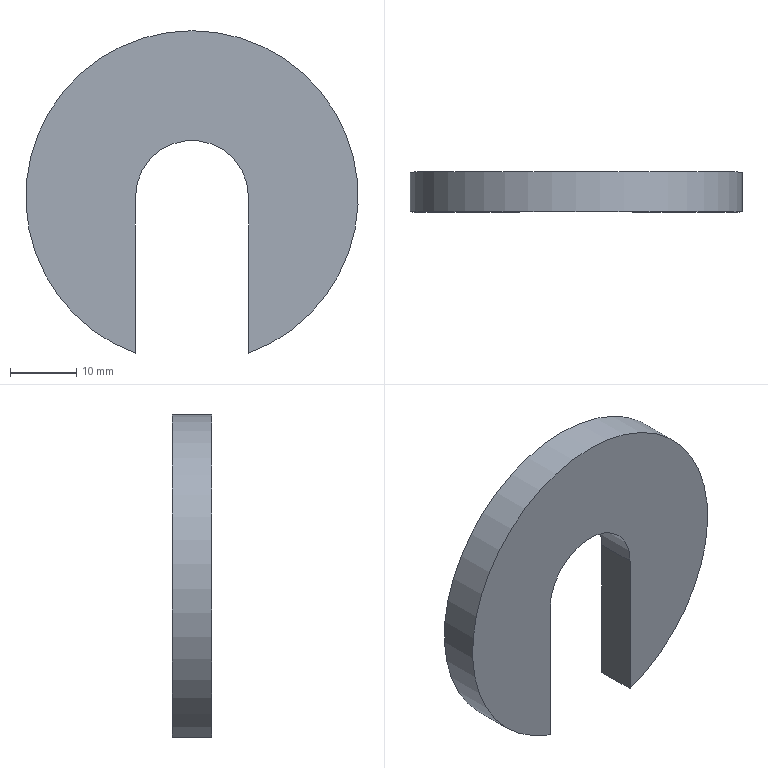Component | NX | C_WASHER | 1 solid | 6 faces | box 50 x 6 x 48.51 mm | volume 8600 mm3 | plane 4 | cylinder 2 | commonest cylinder face diameters 17 x1 50 x1
STEP:
#1=CARTESIAN_POINT('',(0.,0.,0.));
#2=DIRECTION('',(0.,0.,1.));
#3=DIRECTION('',(1.,0.,0.));
#4=AXIS2_PLACEMENT_3D('',#1,#2,#3);
#5=CARTESIAN_POINT('',(-8.5,-38.,42.489));
#6=VERTEX_POINT('',#5);
#7=CARTESIAN_POINT('',(-8.5,-38.,66.));
#8=VERTEX_POINT('',#7);
#9=CARTESIAN_POINT('',(-8.5,-38.,42.489));
#10=DIRECTION('',(-0.,0.,1.));
#11=VECTOR('',#10,1.);
#12=LINE('',#9,#11);
#13=CARTESIAN_POINT('',(-8.5,-44.,42.489));
#14=DIRECTION('',(-1.,0.,-0.));
#15=DIRECTION('',(0.,0.,-1.));
#16=AXIS2_PLACEMENT_3D('',#13,#14,#15);
#17=PLANE('',#16);
#18=CARTESIAN_POINT('',(0.,-6.));
#19=DIRECTION('',(-1.,0.));
#20=VECTOR('',#19,1.);
#21=LINE('',#18,#20);
#22=(GEOMETRIC_REPRESENTATION_CONTEXT(2)PARAMETRIC_REPRESENTATION_CONTEXT()REPRESENTATION_CONTEXT('',''));
#23=DEFINITIONAL_REPRESENTATION('',(#21),#22);
#24=PCURVE('',#17,#23);
#25=CARTESIAN_POINT('',(0.,-38.,66.));
#26=DIRECTION('',(0.,1.,0.));
#27=DIRECTION('',(0.,0.,1.));
#28=AXIS2_PLACEMENT_3D('',#25,#26,#27);
#29=PLANE('',#28);
#30=CARTESIAN_POINT('',(-23.511,-8.5));
#31=DIRECTION('',(1.,-0.));
#32=VECTOR('',#31,1.);
#33=LINE('',#30,#32);
#34=(GEOMETRIC_REPRESENTATION_CONTEXT(2)PARAMETRIC_REPRESENTATION_CONTEXT()REPRESENTATION_CONTEXT('',''));
#35=DEFINITIONAL_REPRESENTATION('',(#33),#34);
#36=PCURVE('',#29,#35);
#37=SURFACE_CURVE('',#12,(#24,#36),.PCURVE_S1.);
#38=EDGE_CURVE('',#6,#8,#37,.T.);
#39=ORIENTED_EDGE('',*,*,#38,.T.);
#40=CARTESIAN_POINT('',(-8.5,-44.,66.));
#41=VERTEX_POINT('',#40);
#42=CARTESIAN_POINT('',(-8.5,-44.,66.));
#43=DIRECTION('',(0.,1.,0.));
#44=VECTOR('',#43,1.);
#45=LINE('',#42,#44);
#46=CARTESIAN_POINT('',(-23.511,0.));
#47=DIRECTION('',(0.,-1.));
#48=VECTOR('',#47,1.);
#49=LINE('',#46,#48);
#50=(GEOMETRIC_REPRESENTATION_CONTEXT(2)PARAMETRIC_REPRESENTATION_CONTEXT()REPRESENTATION_CONTEXT('',''));
#51=DEFINITIONAL_REPRESENTATION('',(#49),#50);
#52=PCURVE('',#17,#51);
#53=CARTESIAN_POINT('',(0.,-44.,66.));
#54=DIRECTION('',(0.,1.,0.));
#55=DIRECTION('',(0.,0.,1.));
#56=AXIS2_PLACEMENT_3D('',#53,#54,#55);
#57=CYLINDRICAL_SURFACE('',#56,8.5);
#58=CARTESIAN_POINT('',(4.712,0.));
#59=DIRECTION('',(0.,1.));
#60=VECTOR('',#59,1.);
#61=LINE('',#58,#60);
#62=(GEOMETRIC_REPRESENTATION_CONTEXT(2)PARAMETRIC_REPRESENTATION_CONTEXT()REPRESENTATION_CONTEXT('',''));
#63=DEFINITIONAL_REPRESENTATION('',(#61),#62);
#64=PCURVE('',#57,#63);
#65=SURFACE_CURVE('',#45,(#52,#64),.PCURVE_S1.);
#66=EDGE_CURVE('',#41,#8,#65,.T.);
#67=ORIENTED_EDGE('',*,*,#66,.F.);
#68=CARTESIAN_POINT('',(-8.5,-44.,42.489));
#69=VERTEX_POINT('',#68);
#70=CARTESIAN_POINT('',(-8.5,-44.,42.489));
#71=DIRECTION('',(-0.,0.,1.));
#72=VECTOR('',#71,1.);
#73=LINE('',#70,#72);
#74=CARTESIAN_POINT('',(0.,0.));
#75=DIRECTION('',(-1.,0.));
#76=VECTOR('',#75,1.);
#77=LINE('',#74,#76);
#78=(GEOMETRIC_REPRESENTATION_CONTEXT(2)PARAMETRIC_REPRESENTATION_CONTEXT()REPRESENTATION_CONTEXT('',''));
#79=DEFINITIONAL_REPRESENTATION('',(#77),#78);
#80=PCURVE('',#17,#79);
#81=CARTESIAN_POINT('',(0.,-44.,66.));
#82=DIRECTION('',(0.,1.,0.));
#83=DIRECTION('',(0.,0.,1.));
#84=AXIS2_PLACEMENT_3D('',#81,#82,#83);
#85=PLANE('',#84);
#86=CARTESIAN_POINT('',(-23.511,-8.5));
#87=DIRECTION('',(1.,-0.));
#88=VECTOR('',#87,1.);
#89=LINE('',#86,#88);
#90=(GEOMETRIC_REPRESENTATION_CONTEXT(2)PARAMETRIC_REPRESENTATION_CONTEXT()REPRESENTATION_CONTEXT('',''));
#91=DEFINITIONAL_REPRESENTATION('',(#89),#90);
#92=PCURVE('',#85,#91);
#93=SURFACE_CURVE('',#73,(#80,#92),.PCURVE_S1.);
#94=EDGE_CURVE('',#69,#41,#93,.T.);
#95=ORIENTED_EDGE('',*,*,#94,.F.);
#96=CARTESIAN_POINT('',(-8.5,-44.,42.489));
#97=DIRECTION('',(0.,1.,0.));
#98=VECTOR('',#97,1.);
#99=LINE('',#96,#98);
#100=CARTESIAN_POINT('',(0.,0.));
#101=DIRECTION('',(0.,-1.));
#102=VECTOR('',#101,1.);
#103=LINE('',#100,#102);
#104=(GEOMETRIC_REPRESENTATION_CONTEXT(2)PARAMETRIC_REPRESENTATION_CONTEXT()REPRESENTATION_CONTEXT('',''));
#105=DEFINITIONAL_REPRESENTATION('',(#103),#104);
#106=PCURVE('',#17,#105);
#107=CARTESIAN_POINT('',(0.,-44.,66.));
#108=DIRECTION('',(0.,1.,0.));
#109=DIRECTION('',(0.,0.,1.));
#110=AXIS2_PLACEMENT_3D('',#107,#108,#109);
#111=CYLINDRICAL_SURFACE('',#110,25.);
#112=CARTESIAN_POINT('',(3.489,0.));
#113=DIRECTION('',(0.,1.));
#114=VECTOR('',#113,1.);
#115=LINE('',#112,#114);
#116=(GEOMETRIC_REPRESENTATION_CONTEXT(2)PARAMETRIC_REPRESENTATION_CONTEXT()REPRESENTATION_CONTEXT('',''));
#117=DEFINITIONAL_REPRESENTATION('',(#115),#116);
#118=PCURVE('',#111,#117);
#119=SURFACE_CURVE('',#99,(#106,#118),.PCURVE_S1.);
#120=EDGE_CURVE('',#69,#6,#119,.T.);
#121=ORIENTED_EDGE('',*,*,#120,.T.);
#122=EDGE_LOOP('',(#39,#67,#95,#121));
#123=FACE_BOUND('',#122,.T.);
#124=ADVANCED_FACE('',(#123),#17,.F.);
#125=ORIENTED_EDGE('',*,*,#66,.F.);
#126=CARTESIAN_POINT('',(8.5,-44.,66.));
#127=VERTEX_POINT('',#126);
#128=CARTESIAN_POINT('',(0.,-44.,66.));
#129=DIRECTION('',(0.,1.,0.));
#130=DIRECTION('',(1.,0.,0.));
#131=AXIS2_PLACEMENT_3D('',#128,#129,#130);
#132=CIRCLE('',#131,8.5);
#133=CARTESIAN_POINT('',(1.571,0.));
#134=DIRECTION('',(1.,0.));
#135=VECTOR('',#134,1.);
#136=LINE('',#133,#135);
#137=(GEOMETRIC_REPRESENTATION_CONTEXT(2)PARAMETRIC_REPRESENTATION_CONTEXT()REPRESENTATION_CONTEXT('',''));
#138=DEFINITIONAL_REPRESENTATION('',(#136),#137);
#139=PCURVE('',#57,#138);
#140=CARTESIAN_POINT('',(0.,0.));
#141=DIRECTION('',(0.,1.));
#142=AXIS2_PLACEMENT_2D('',#140,#141);
#143=CIRCLE('',#142,8.5);
#144=(GEOMETRIC_REPRESENTATION_CONTEXT(2)PARAMETRIC_REPRESENTATION_CONTEXT()REPRESENTATION_CONTEXT('',''));
#145=DEFINITIONAL_REPRESENTATION('',(#143),#144);
#146=PCURVE('',#85,#145);
#147=SURFACE_CURVE('',#132,(#139,#146),.PCURVE_S1.);
#148=EDGE_CURVE('',#41,#127,#147,.T.);
#149=ORIENTED_EDGE('',*,*,#148,.T.);
#150=CARTESIAN_POINT('',(8.5,-38.,66.));
#151=VERTEX_POINT('',#150);
#152=CARTESIAN_POINT('',(8.5,-44.,66.));
#153=DIRECTION('',(0.,1.,0.));
#154=VECTOR('',#153,1.);
#155=LINE('',#152,#154);
#156=CARTESIAN_POINT('',(7.854,0.));
#157=DIRECTION('',(0.,1.));
#158=VECTOR('',#157,1.);
#159=LINE('',#156,#158);
#160=(GEOMETRIC_REPRESENTATION_CONTEXT(2)PARAMETRIC_REPRESENTATION_CONTEXT()REPRESENTATION_CONTEXT('',''));
#161=DEFINITIONAL_REPRESENTATION('',(#159),#160);
#162=PCURVE('',#57,#161);
#163=CARTESIAN_POINT('',(8.5,-44.,66.));
#164=DIRECTION('',(1.,0.,0.));
#165=DIRECTION('',(-0.,0.,1.));
#166=AXIS2_PLACEMENT_3D('',#163,#164,#165);
#167=PLANE('',#166);
#168=CARTESIAN_POINT('',(0.,0.));
#169=DIRECTION('',(0.,-1.));
#170=VECTOR('',#169,1.);
#171=LINE('',#168,#170);
#172=(GEOMETRIC_REPRESENTATION_CONTEXT(2)PARAMETRIC_REPRESENTATION_CONTEXT()REPRESENTATION_CONTEXT('',''));
#173=DEFINITIONAL_REPRESENTATION('',(#171),#172);
#174=PCURVE('',#167,#173);
#175=SURFACE_CURVE('',#155,(#162,#174),.PCURVE_S1.);
#176=EDGE_CURVE('',#127,#151,#175,.T.);
#177=ORIENTED_EDGE('',*,*,#176,.T.);
#178=CARTESIAN_POINT('',(0.,-38.,66.));
#179=DIRECTION('',(0.,1.,0.));
#180=DIRECTION('',(1.,0.,0.));
#181=AXIS2_PLACEMENT_3D('',#178,#179,#180);
#182=CIRCLE('',#181,8.5);
#183=CARTESIAN_POINT('',(1.571,6.));
#184=DIRECTION('',(1.,0.));
#185=VECTOR('',#184,1.);
#186=LINE('',#183,#185);
#187=(GEOMETRIC_REPRESENTATION_CONTEXT(2)PARAMETRIC_REPRESENTATION_CONTEXT()REPRESENTATION_CONTEXT('',''));
#188=DEFINITIONAL_REPRESENTATION('',(#186),#187);
#189=PCURVE('',#57,#188);
#190=CARTESIAN_POINT('',(0.,0.));
#191=DIRECTION('',(0.,1.));
#192=AXIS2_PLACEMENT_2D('',#190,#191);
#193=CIRCLE('',#192,8.5);
#194=(GEOMETRIC_REPRESENTATION_CONTEXT(2)PARAMETRIC_REPRESENTATION_CONTEXT()REPRESENTATION_CONTEXT('',''));
#195=DEFINITIONAL_REPRESENTATION('',(#193),#194);
#196=PCURVE('',#29,#195);
#197=SURFACE_CURVE('',#182,(#189,#196),.PCURVE_S1.);
#198=EDGE_CURVE('',#8,#151,#197,.T.);
#199=ORIENTED_EDGE('',*,*,#198,.F.);
#200=EDGE_LOOP('',(#125,#149,#177,#199));
#201=FACE_BOUND('',#200,.F.);
#202=ADVANCED_FACE('',(#201),#57,.F.);
#203=CARTESIAN_POINT('',(8.5,-38.,42.489));
#204=VERTEX_POINT('',#203);
#205=CARTESIAN_POINT('',(8.5,-38.,66.));
#206=DIRECTION('',(0.,0.,-1.));
#207=VECTOR('',#206,1.);
#208=LINE('',#205,#207);
#209=CARTESIAN_POINT('',(0.,-6.));
#210=DIRECTION('',(-1.,0.));
#211=VECTOR('',#210,1.);
#212=LINE('',#209,#211);
#213=(GEOMETRIC_REPRESENTATION_CONTEXT(2)PARAMETRIC_REPRESENTATION_CONTEXT()REPRESENTATION_CONTEXT('',''));
#214=DEFINITIONAL_REPRESENTATION('',(#212),#213);
#215=PCURVE('',#167,#214);
#216=CARTESIAN_POINT('',(0.,8.5));
#217=DIRECTION('',(-1.,0.));
#218=VECTOR('',#217,1.);
#219=LINE('',#216,#218);
#220=(GEOMETRIC_REPRESENTATION_CONTEXT(2)PARAMETRIC_REPRESENTATION_CONTEXT()REPRESENTATION_CONTEXT('',''));
#221=DEFINITIONAL_REPRESENTATION('',(#219),#220);
#222=PCURVE('',#29,#221);
#223=SURFACE_CURVE('',#208,(#215,#222),.PCURVE_S1.);
#224=EDGE_CURVE('',#151,#204,#223,.T.);
#225=ORIENTED_EDGE('',*,*,#224,.T.);
#226=CARTESIAN_POINT('',(8.5,-44.,42.489));
#227=VERTEX_POINT('',#226);
#228=CARTESIAN_POINT('',(8.5,-44.,42.489));
#229=DIRECTION('',(0.,1.,0.));
#230=VECTOR('',#229,1.);
#231=LINE('',#228,#230);
#232=CARTESIAN_POINT('',(-23.511,0.));
#233=DIRECTION('',(0.,-1.));
#234=VECTOR('',#233,1.);
#235=LINE('',#232,#234);
#236=(GEOMETRIC_REPRESENTATION_CONTEXT(2)PARAMETRIC_REPRESENTATION_CONTEXT()REPRESENTATION_CONTEXT('',''));
#237=DEFINITIONAL_REPRESENTATION('',(#235),#236);
#238=PCURVE('',#167,#237);
#239=CARTESIAN_POINT('',(9.078,0.));
#240=DIRECTION('',(0.,1.));
#241=VECTOR('',#240,1.);
#242=LINE('',#239,#241);
#243=(GEOMETRIC_REPRESENTATION_CONTEXT(2)PARAMETRIC_REPRESENTATION_CONTEXT()REPRESENTATION_CONTEXT('',''));
#244=DEFINITIONAL_REPRESENTATION('',(#242),#243);
#245=PCURVE('',#111,#244);
#246=SURFACE_CURVE('',#231,(#238,#245),.PCURVE_S1.);
#247=EDGE_CURVE('',#227,#204,#246,.T.);
#248=ORIENTED_EDGE('',*,*,#247,.F.);
#249=CARTESIAN_POINT('',(8.5,-44.,66.));
#250=DIRECTION('',(0.,0.,-1.));
#251=VECTOR('',#250,1.);
#252=LINE('',#249,#251);
#253=CARTESIAN_POINT('',(0.,0.));
#254=DIRECTION('',(-1.,0.));
#255=VECTOR('',#254,1.);
#256=LINE('',#253,#255);
#257=(GEOMETRIC_REPRESENTATION_CONTEXT(2)PARAMETRIC_REPRESENTATION_CONTEXT()REPRESENTATION_CONTEXT('',''));
#258=DEFINITIONAL_REPRESENTATION('',(#256),#257);
#259=PCURVE('',#167,#258);
#260=CARTESIAN_POINT('',(0.,8.5));
#261=DIRECTION('',(-1.,0.));
#262=VECTOR('',#261,1.);
#263=LINE('',#260,#262);
#264=(GEOMETRIC_REPRESENTATION_CONTEXT(2)PARAMETRIC_REPRESENTATION_CONTEXT()REPRESENTATION_CONTEXT('',''));
#265=DEFINITIONAL_REPRESENTATION('',(#263),#264);
#266=PCURVE('',#85,#265);
#267=SURFACE_CURVE('',#252,(#259,#266),.PCURVE_S1.);
#268=EDGE_CURVE('',#127,#227,#267,.T.);
#269=ORIENTED_EDGE('',*,*,#268,.F.);
#270=ORIENTED_EDGE('',*,*,#176,.T.);
#271=EDGE_LOOP('',(#225,#248,#269,#270));
#272=FACE_BOUND('',#271,.T.);
#273=ADVANCED_FACE('',(#272),#167,.F.);
#274=CARTESIAN_POINT('',(0.,-38.,66.));
#275=DIRECTION('',(0.,-1.,0.));
#276=DIRECTION('',(1.,0.,0.));
#277=AXIS2_PLACEMENT_3D('',#274,#275,#276);
#278=CIRCLE('',#277,25.);
#279=CARTESIAN_POINT('',(14.137,6.));
#280=DIRECTION('',(-1.,0.));
#281=VECTOR('',#280,1.);
#282=LINE('',#279,#281);
#283=(GEOMETRIC_REPRESENTATION_CONTEXT(2)PARAMETRIC_REPRESENTATION_CONTEXT()REPRESENTATION_CONTEXT('',''));
#284=DEFINITIONAL_REPRESENTATION('',(#282),#283);
#285=PCURVE('',#111,#284);
#286=CARTESIAN_POINT('',(0.,25.));
#287=CARTESIAN_POINT('',(43.301,25.));
#288=CARTESIAN_POINT('',(21.651,-12.5));
#289=CARTESIAN_POINT('',(0.,-50.));
#290=CARTESIAN_POINT('',(-21.651,-12.5));
#291=CARTESIAN_POINT('',(-43.301,25.));
#292=CARTESIAN_POINT('',(0.,25.));
#293=(BOUNDED_CURVE()B_SPLINE_CURVE(2,(#286,#287,#288,#289,#290,#291,#292),.UNSPECIFIED.,.T.,.F.)B_SPLINE_CURVE_WITH_KNOTS((1,2,2,2,2,1),(-2.094,0.,2.094,4.189,6.283,8.378),.UNSPECIFIED.)CURVE()GEOMETRIC_REPRESENTATION_ITEM()RATIONAL_B_SPLINE_CURVE((1.,0.5,1.,0.5,1.,0.5,1.))REPRESENTATION_ITEM(''));
#294=(GEOMETRIC_REPRESENTATION_CONTEXT(2)PARAMETRIC_REPRESENTATION_CONTEXT()REPRESENTATION_CONTEXT('',''));
#295=DEFINITIONAL_REPRESENTATION('',(#293),#294);
#296=PCURVE('',#29,#295);
#297=SURFACE_CURVE('',#278,(#285,#296),.PCURVE_S1.);
#298=EDGE_CURVE('',#204,#6,#297,.T.);
#299=ORIENTED_EDGE('',*,*,#298,.T.);
#300=ORIENTED_EDGE('',*,*,#120,.F.);
#301=CARTESIAN_POINT('',(0.,-44.,66.));
#302=DIRECTION('',(0.,-1.,0.));
#303=DIRECTION('',(1.,0.,0.));
#304=AXIS2_PLACEMENT_3D('',#301,#302,#303);
#305=CIRCLE('',#304,25.);
#306=CARTESIAN_POINT('',(14.137,0.));
#307=DIRECTION('',(-1.,0.));
#308=VECTOR('',#307,1.);
#309=LINE('',#306,#308);
#310=(GEOMETRIC_REPRESENTATION_CONTEXT(2)PARAMETRIC_REPRESENTATION_CONTEXT()REPRESENTATION_CONTEXT('',''));
#311=DEFINITIONAL_REPRESENTATION('',(#309),#310);
#312=PCURVE('',#111,#311);
#313=CARTESIAN_POINT('',(0.,25.));
#314=CARTESIAN_POINT('',(43.301,25.));
#315=CARTESIAN_POINT('',(21.651,-12.5));
#316=CARTESIAN_POINT('',(0.,-50.));
#317=CARTESIAN_POINT('',(-21.651,-12.5));
#318=CARTESIAN_POINT('',(-43.301,25.));
#319=CARTESIAN_POINT('',(0.,25.));
#320=(BOUNDED_CURVE()B_SPLINE_CURVE(2,(#313,#314,#315,#316,#317,#318,#319),.UNSPECIFIED.,.T.,.F.)B_SPLINE_CURVE_WITH_KNOTS((1,2,2,2,2,1),(-2.094,0.,2.094,4.189,6.283,8.378),.UNSPECIFIED.)CURVE()GEOMETRIC_REPRESENTATION_ITEM()RATIONAL_B_SPLINE_CURVE((1.,0.5,1.,0.5,1.,0.5,1.))REPRESENTATION_ITEM(''));
#321=(GEOMETRIC_REPRESENTATION_CONTEXT(2)PARAMETRIC_REPRESENTATION_CONTEXT()REPRESENTATION_CONTEXT('',''));
#322=DEFINITIONAL_REPRESENTATION('',(#320),#321);
#323=PCURVE('',#85,#322);
#324=SURFACE_CURVE('',#305,(#312,#323),.PCURVE_S1.);
#325=EDGE_CURVE('',#227,#69,#324,.T.);
#326=ORIENTED_EDGE('',*,*,#325,.F.);
#327=ORIENTED_EDGE('',*,*,#247,.T.);
#328=EDGE_LOOP('',(#299,#300,#326,#327));
#329=FACE_BOUND('',#328,.T.);
#330=ADVANCED_FACE('',(#329),#111,.T.);
#331=ORIENTED_EDGE('',*,*,#94,.T.);
#332=ORIENTED_EDGE('',*,*,#148,.T.);
#333=ORIENTED_EDGE('',*,*,#268,.T.);
#334=ORIENTED_EDGE('',*,*,#325,.T.);
#335=EDGE_LOOP('',(#331,#332,#333,#334));
#336=FACE_BOUND('',#335,.T.);
#337=ADVANCED_FACE('',(#336),#85,.F.);
#338=ORIENTED_EDGE('',*,*,#38,.F.);
#339=ORIENTED_EDGE('',*,*,#298,.F.);
#340=ORIENTED_EDGE('',*,*,#224,.F.);
#341=ORIENTED_EDGE('',*,*,#198,.F.);
#342=EDGE_LOOP('',(#338,#339,#340,#341));
#343=FACE_BOUND('',#342,.T.);
#344=ADVANCED_FACE('',(#343),#29,.T.);
#345=CLOSED_SHELL('',(#124,#202,#273,#330,#337,#344));
#346=MANIFOLD_SOLID_BREP('',#345);
#347=(LENGTH_UNIT()NAMED_UNIT(*)SI_UNIT(.MILLI.,.METRE.));
#348=UNCERTAINTY_MEASURE_WITH_UNIT(LENGTH_MEASURE(0.0000001),#347,'','');
#349=(NAMED_UNIT(*)PLANE_ANGLE_UNIT()SI_UNIT($,.RADIAN.));
#350=(NAMED_UNIT(*)SI_UNIT($,.STERADIAN.)SOLID_ANGLE_UNIT());
#351=(GEOMETRIC_REPRESENTATION_CONTEXT(3)GLOBAL_UNCERTAINTY_ASSIGNED_CONTEXT((#348))GLOBAL_UNIT_ASSIGNED_CONTEXT((#347,#349,#350))REPRESENTATION_CONTEXT('',''));
#352=ADVANCED_BREP_SHAPE_REPRESENTATION('',(#4,#346),#351);